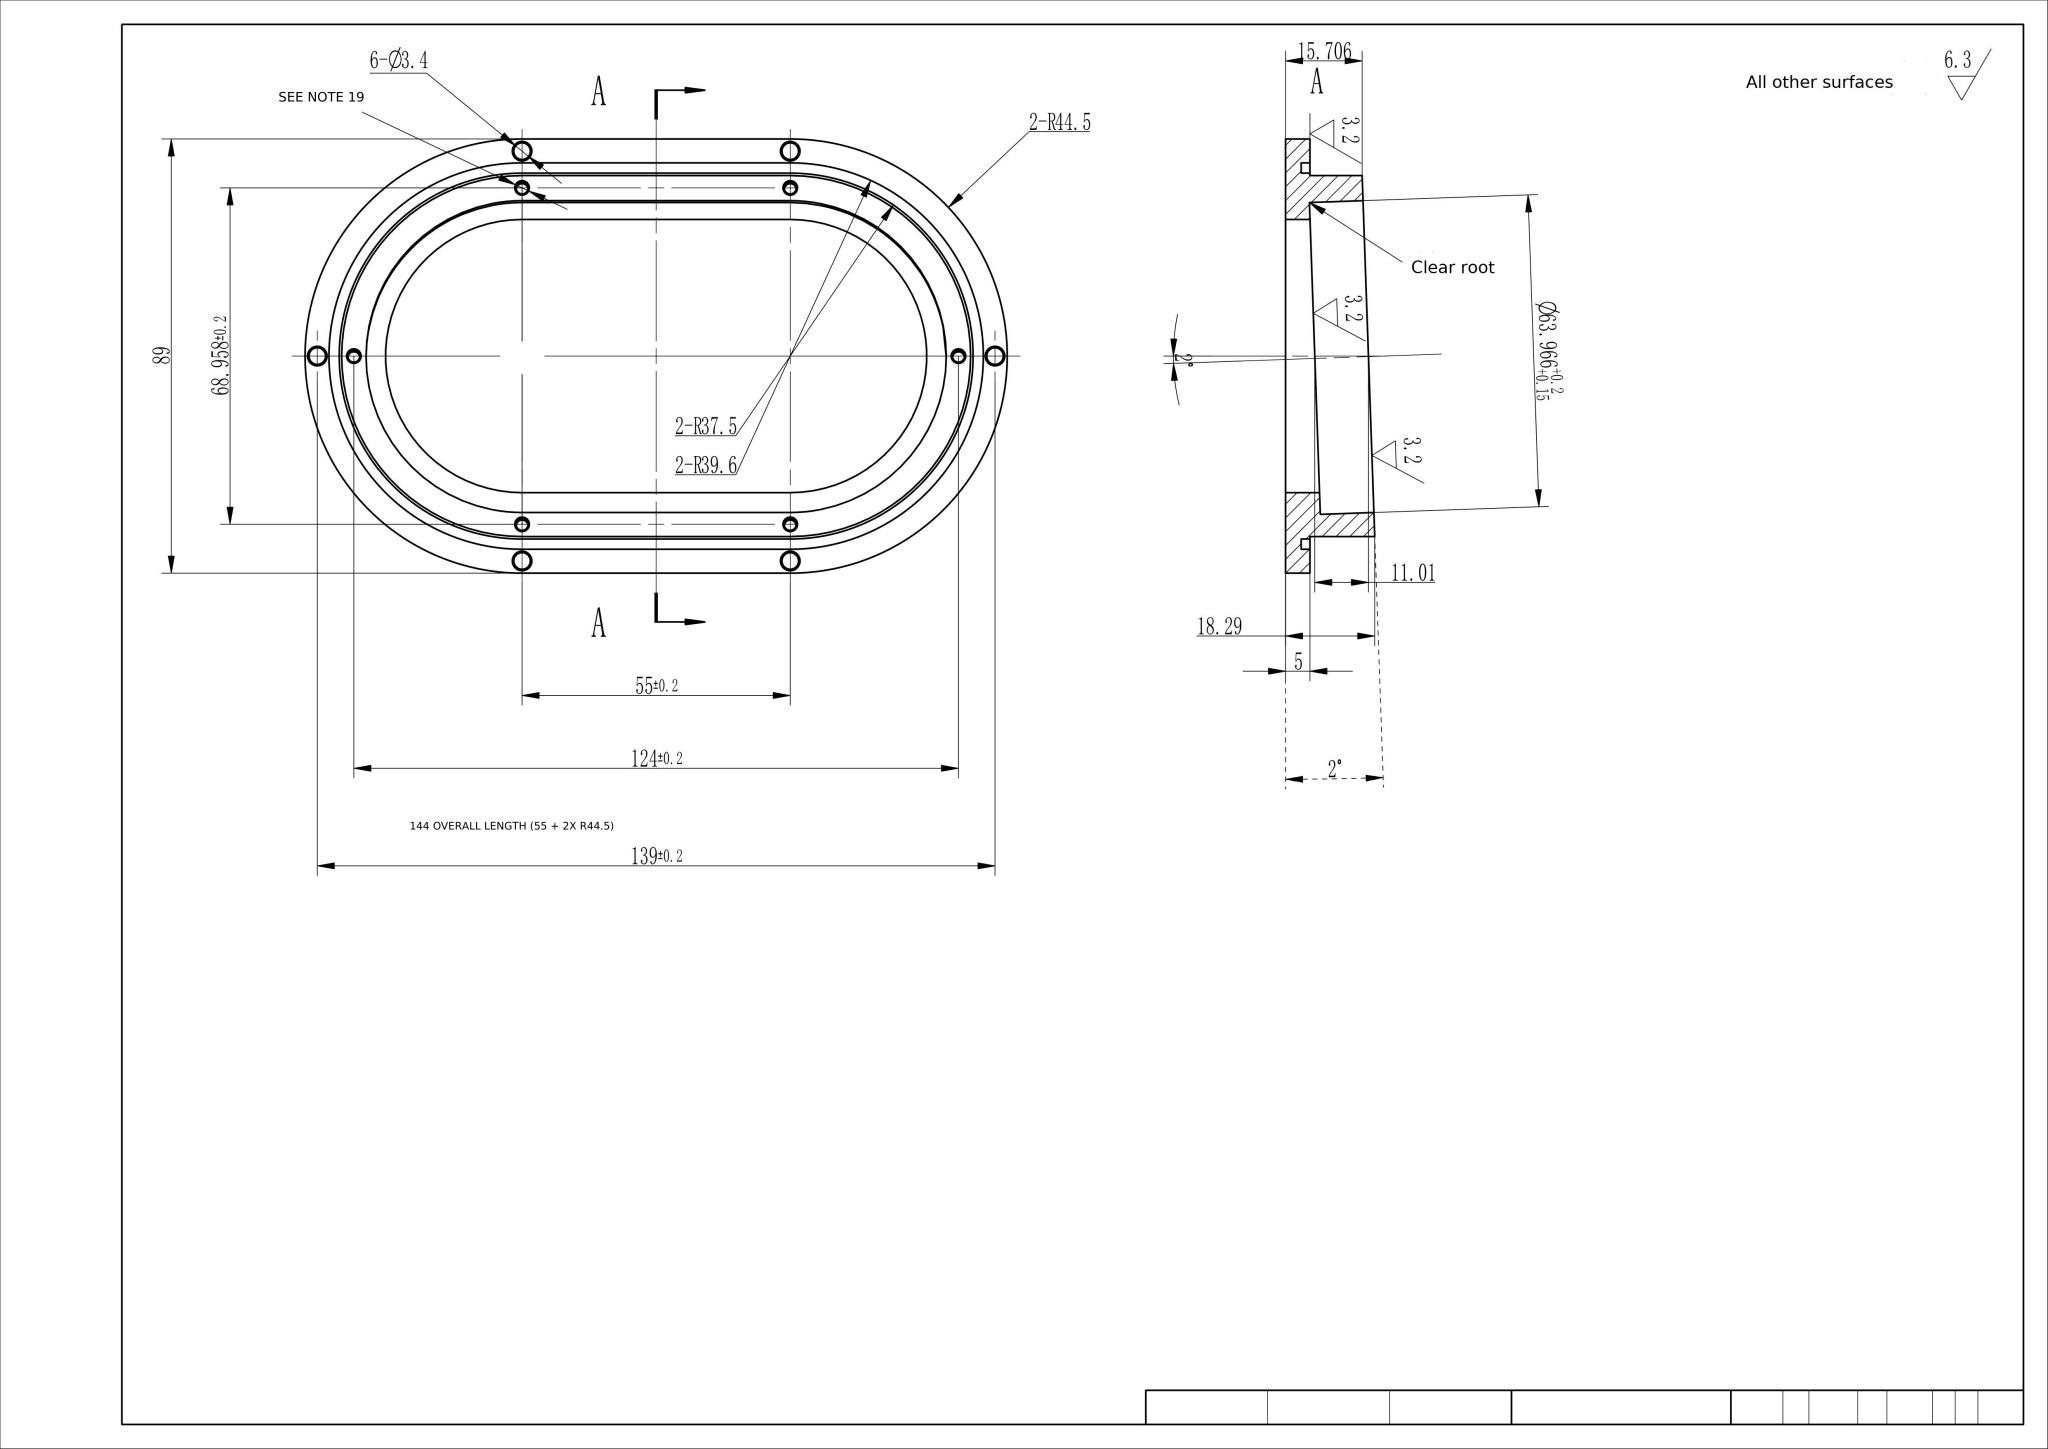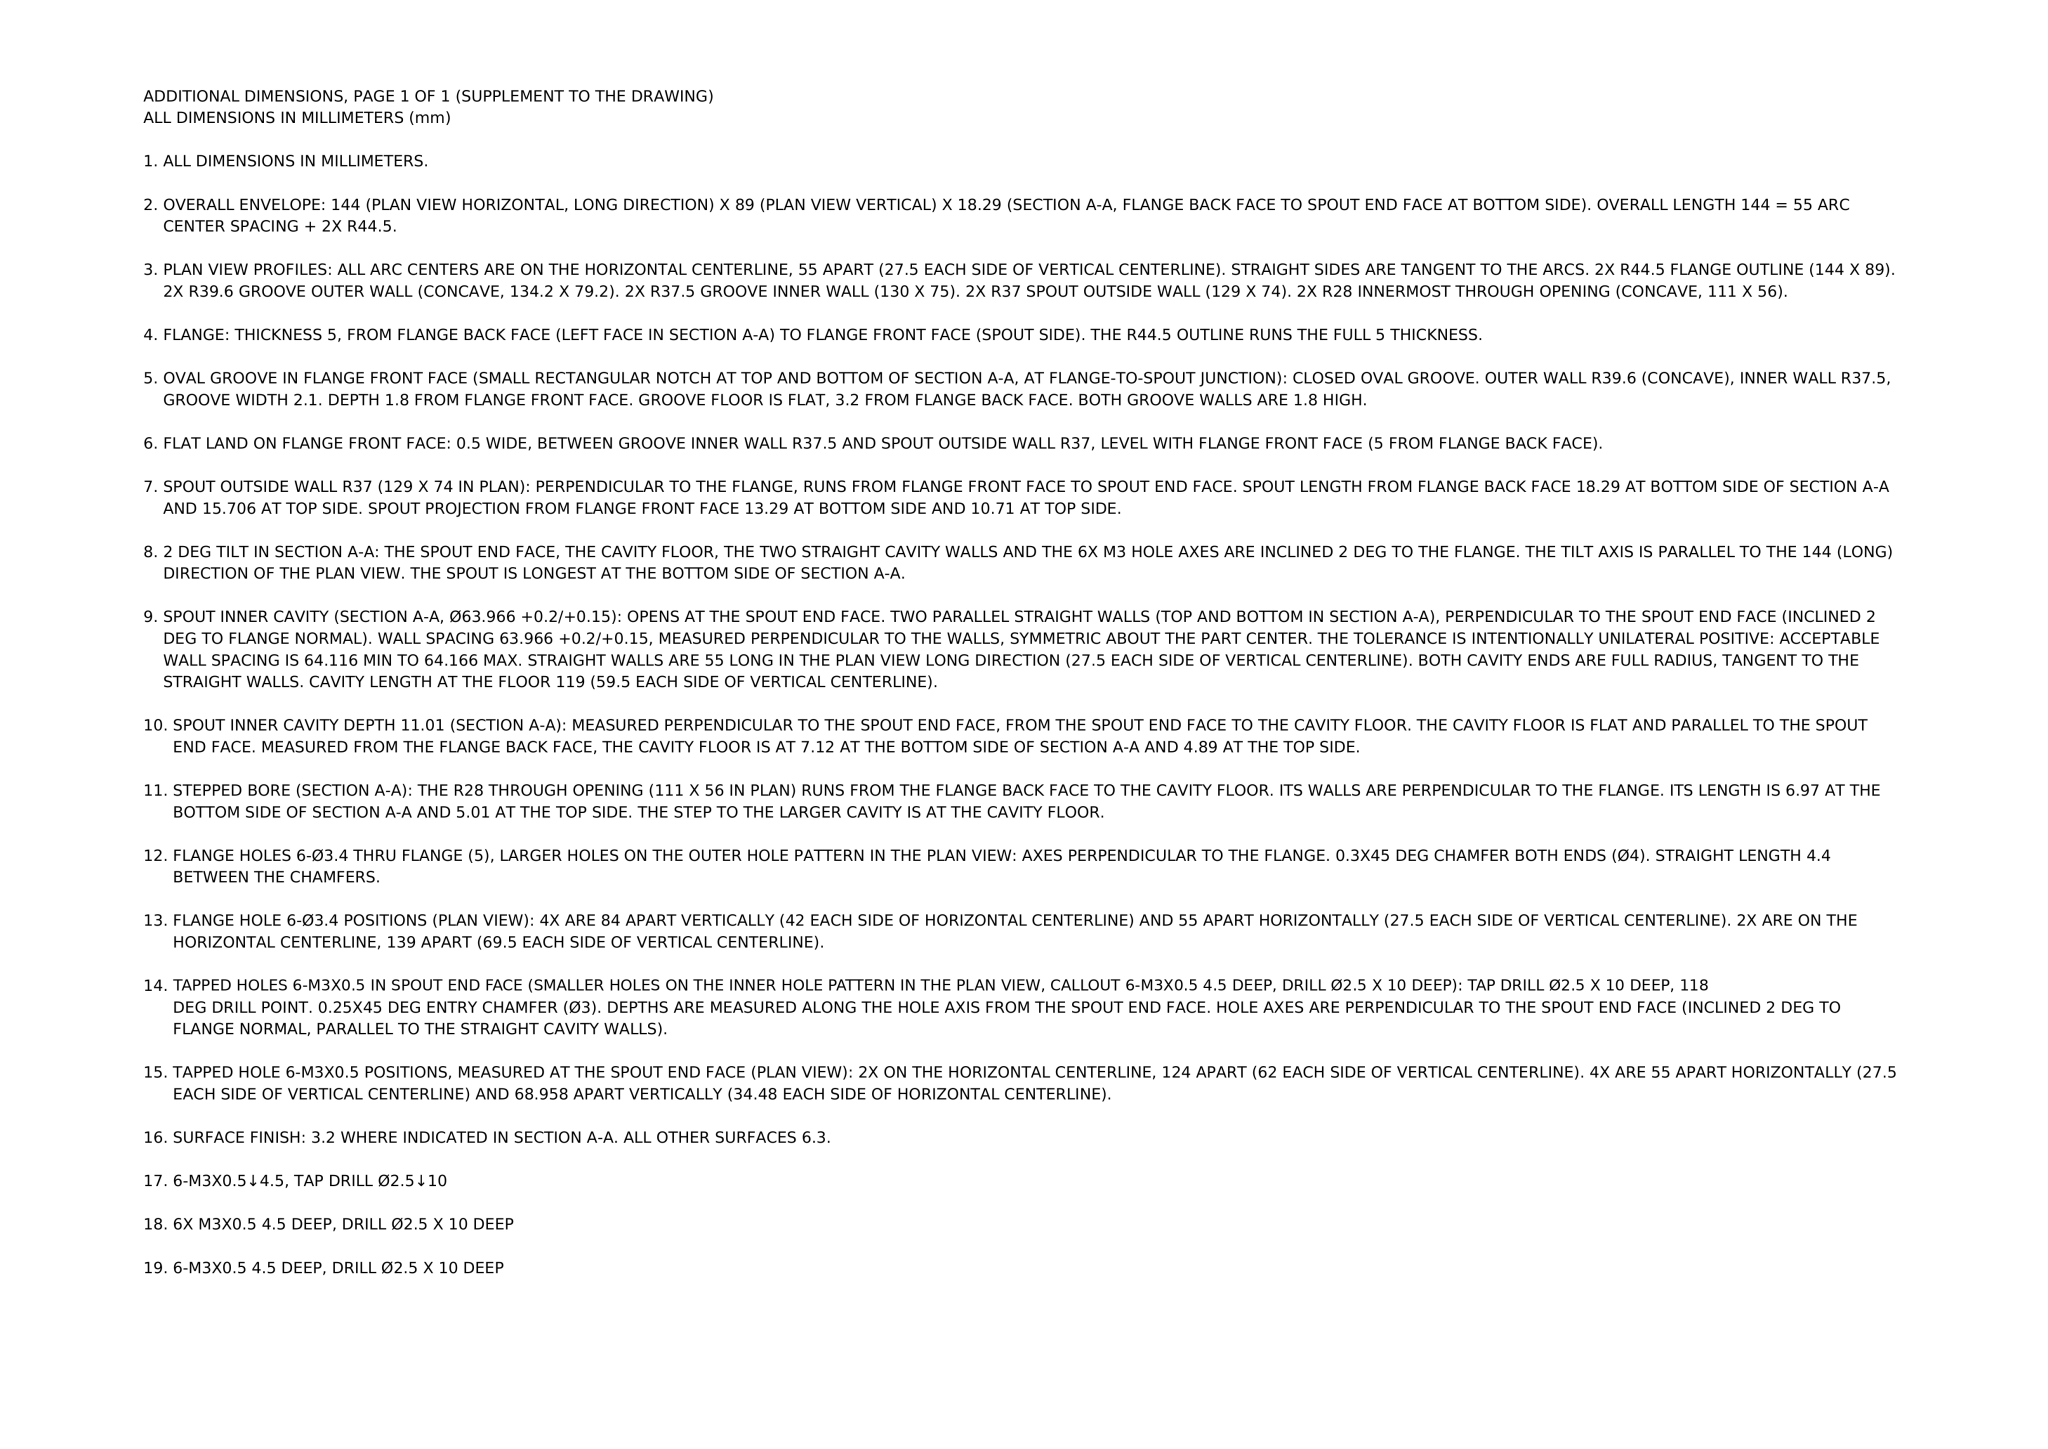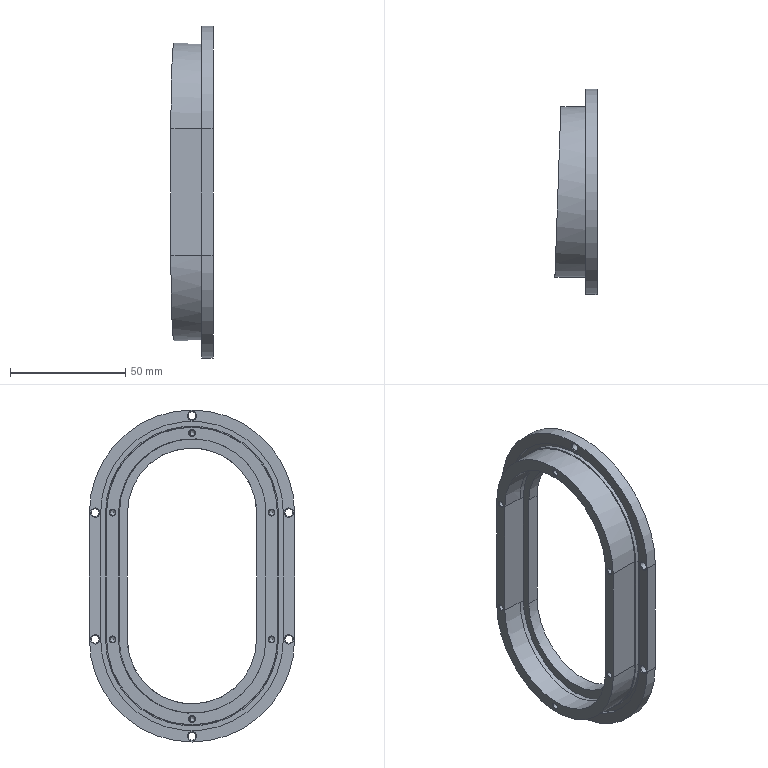Part | NX | mm | 1 solid | 68 faces | box 18.29 x 89 x 144 mm | volume 46824 mm3 | cone 24 | cylinder 22 | plane 18 | other 4 | commonest cylinder face diameters 3.4 x6 2.5 x6 56 x2 74 x2 89 x2 75 x2 79.2 x2